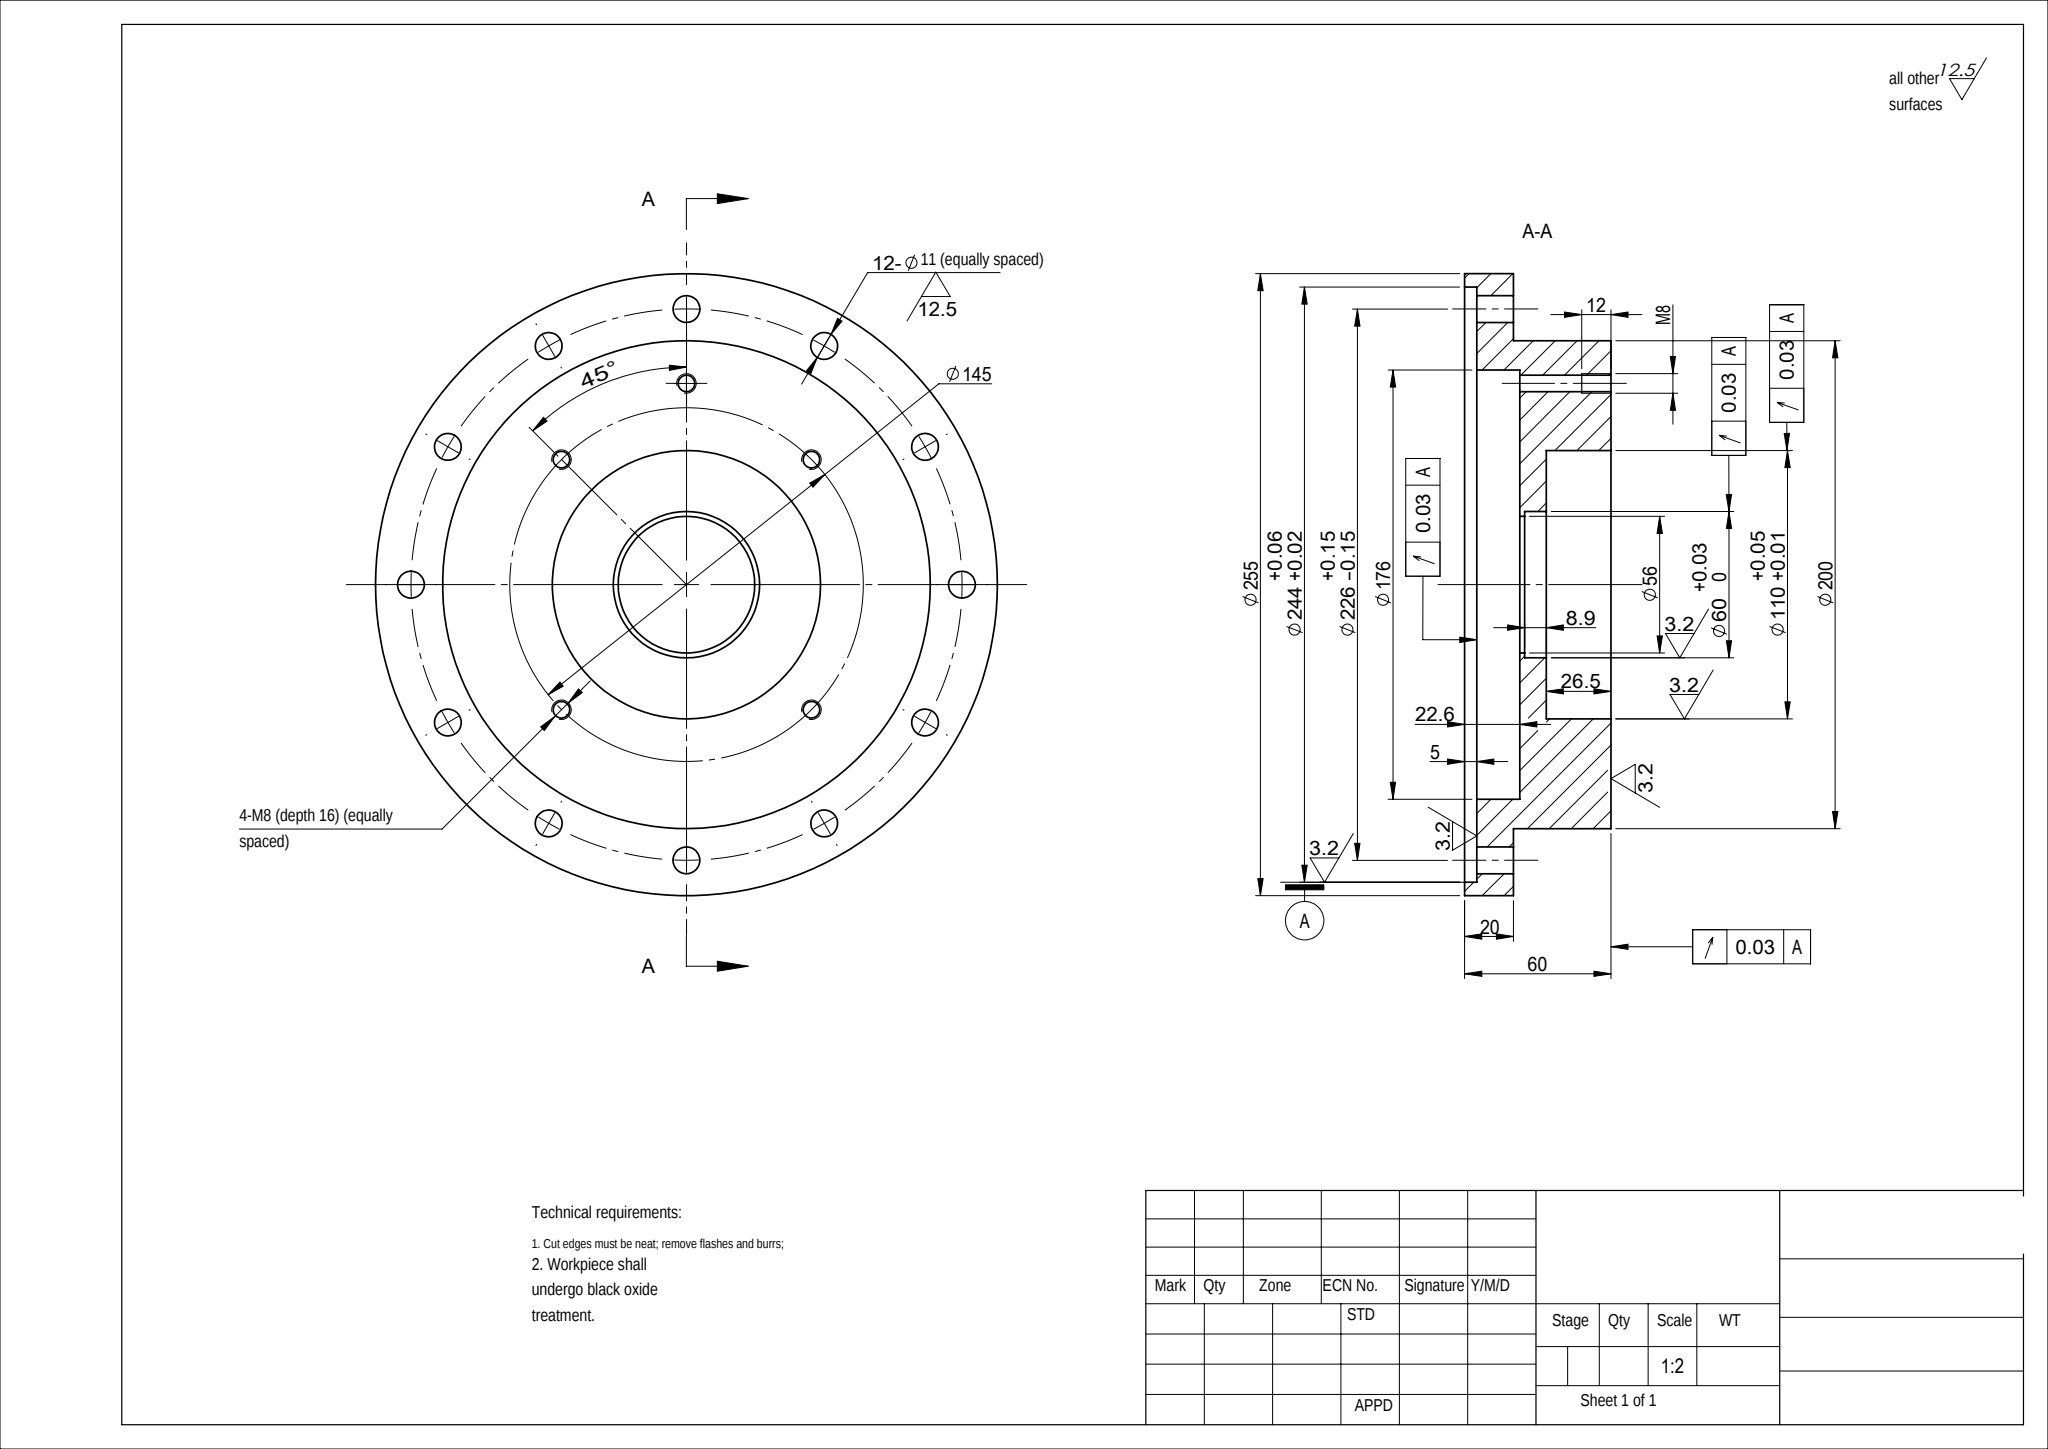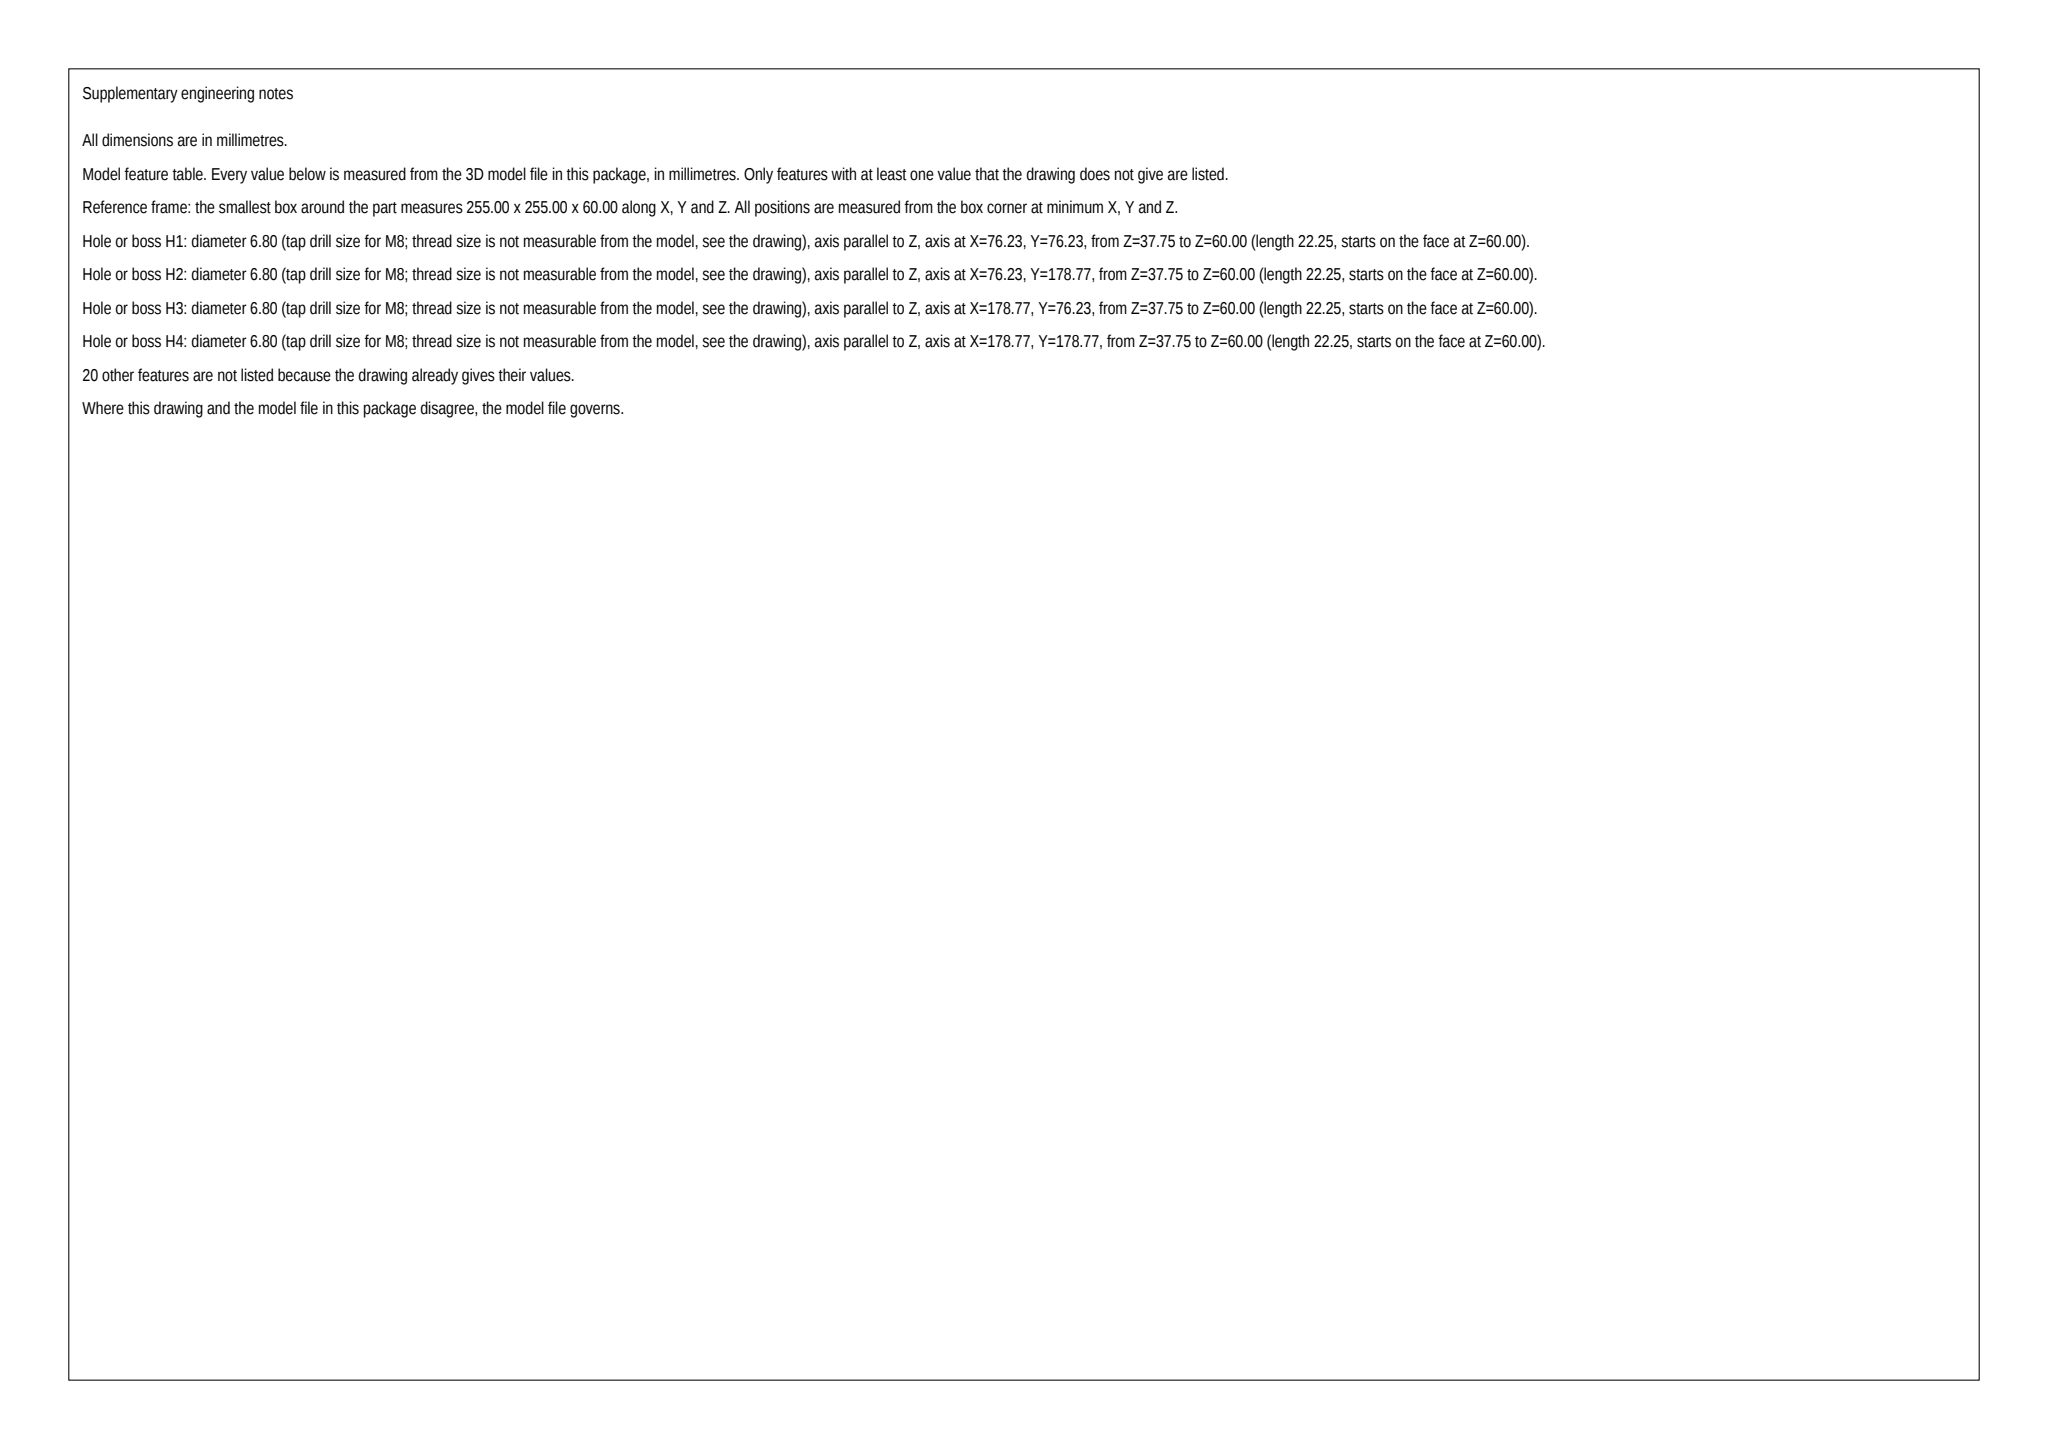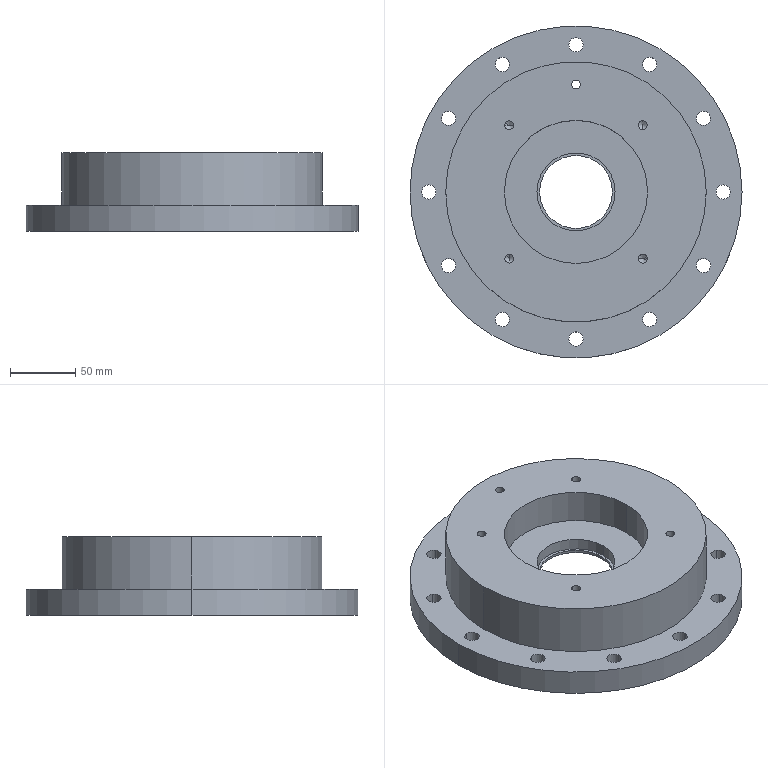Part | SolidWorks | mm | 1 solid | 63 faces | box 255 x 255 x 60 mm | volume 1312345 mm3 | cylinder 48 | cone 8 | plane 7 | commonest cylinder face diameters 11 x24 6.8 x10 176 x2 244 x2 60 x2 110 x2 200 x2 255 x2
build123d program:
from build123d import *

# Parameters (mm, degrees)
SKETCH1_R           = 127.5
BOSS_EXTRUDE1_DEPTH = 20
SKETCH2_R           = 100
BOSS_EXTRUDE2_DEPTH = 40
SKETCH3_R           = 55
CUT_EXTRUDE1_DEPTH  = 26.5
SKETCH4_R           = 28
CUT_EXTRUDE2_DEPTH  = 184.398
SKETCH5_R           = 30
CUT_EXTRUDE3_DEPTH  = 8.9
SKETCH6_R           = 122
CUT_EXTRUDE4_DEPTH  = 5
SKETCH7_R           = 88
CUT_EXTRUDE5_DEPTH  = 17.6
SKETCH8_R           = 5.5
CUT_EXTRUDE6_DEPTH  = 185.696
CIRPATTERN1_COUNT   = 12
SKETCH9_R           = 3.4
CUT_EXTRUDE7_DEPTH  = 191.033
CIRPATTERN2_COUNT   = 4


with BuildPart() as part:
    # Sketch1 → Boss-Extrude1 (new body)
    with BuildSketch(Plane.XY):
        Circle(SKETCH1_R)
    extrude(amount=BOSS_EXTRUDE1_DEPTH)

    # Sketch2 → Boss-Extrude2 (add)
    with BuildSketch(Plane.XY.offset(20)):
        Circle(SKETCH2_R)
    extrude(amount=BOSS_EXTRUDE2_DEPTH)

    # Sketch3 → Cut-Extrude1 (cut)
    with BuildSketch(Plane.XY.offset(60)):
        Circle(SKETCH3_R)
    extrude(amount=-CUT_EXTRUDE1_DEPTH, mode=Mode.SUBTRACT)

    # Sketch4 → Cut-Extrude2 (cut, through all)
    with BuildSketch(Plane.XY.offset(33.5)):
        Circle(SKETCH4_R)
    extrude(amount=-CUT_EXTRUDE2_DEPTH, mode=Mode.SUBTRACT)

    # Sketch5 → Cut-Extrude3 (cut)
    with BuildSketch(Plane.XY.offset(33.5)):
        Circle(SKETCH5_R)
    extrude(amount=-CUT_EXTRUDE3_DEPTH, mode=Mode.SUBTRACT)

    # Sketch6 → Cut-Extrude4 (cut)
    with BuildSketch(Plane(origin=(0, 0, 0), x_dir=(-1, 0, 0), z_dir=(0, 0, -1))):
        Circle(SKETCH6_R)
    extrude(amount=-CUT_EXTRUDE4_DEPTH, mode=Mode.SUBTRACT)

    # Sketch7 → Cut-Extrude5 (cut)
    with BuildSketch(Plane(origin=(0, 0, 5), x_dir=(-1, 0, 0), z_dir=(0, 0, -1))):
        Circle(SKETCH7_R)
    extrude(amount=-CUT_EXTRUDE5_DEPTH, mode=Mode.SUBTRACT)

    # Sketch8 → Cut-Extrude6 (cut, through all)
    with BuildSketch(Plane.XY.offset(20)):
        with Locations((0, 113)):
            Circle(SKETCH8_R)
    cut_extrude6 = extrude(amount=-CUT_EXTRUDE6_DEPTH, mode=Mode.SUBTRACT)

    # CirPattern1: Cut-Extrude6 ×12 about axis
    cirpattern1_axis = Axis((0, 0, 0), (0, 0, 1))
    for i in range(1, CIRPATTERN1_COUNT):
        add(cut_extrude6.rotate(cirpattern1_axis, i * 360 / CIRPATTERN1_COUNT), mode=Mode.SUBTRACT)

    # Sketch9 → Cut-Extrude7 (cut, through all)
    with BuildSketch(Plane.XY.offset(60)):
        with Locations((0, 82.5)):
            Circle(SKETCH9_R)
    extrude(amount=-CUT_EXTRUDE7_DEPTH, mode=Mode.SUBTRACT)

    # Sketch10 → M8 Tapped Hole1 (revolve, cut)
    with BuildSketch(Plane(origin=(-51.265, 51.265, 60), x_dir=(0, -1, 0), z_dir=(1, 0, 0))):
        Polygon((0, 0), (0, 24.293), (3.4, 22.25), (3.4, 0), align=None)
    m8_tapped_hole1 = revolve(axis=Axis((-51.265, 51.265, 66.35), (0, 0, -1)), mode=Mode.SUBTRACT)

    # CirPattern2: M8 Tapped Hole1 ×4 about axis
    cirpattern2_axis = Axis((0, 0, 0), (0, 0, 1))
    for i in range(1, CIRPATTERN2_COUNT):
        add(m8_tapped_hole1.rotate(cirpattern2_axis, i * 360 / CIRPATTERN2_COUNT), mode=Mode.SUBTRACT)


solid = part.part